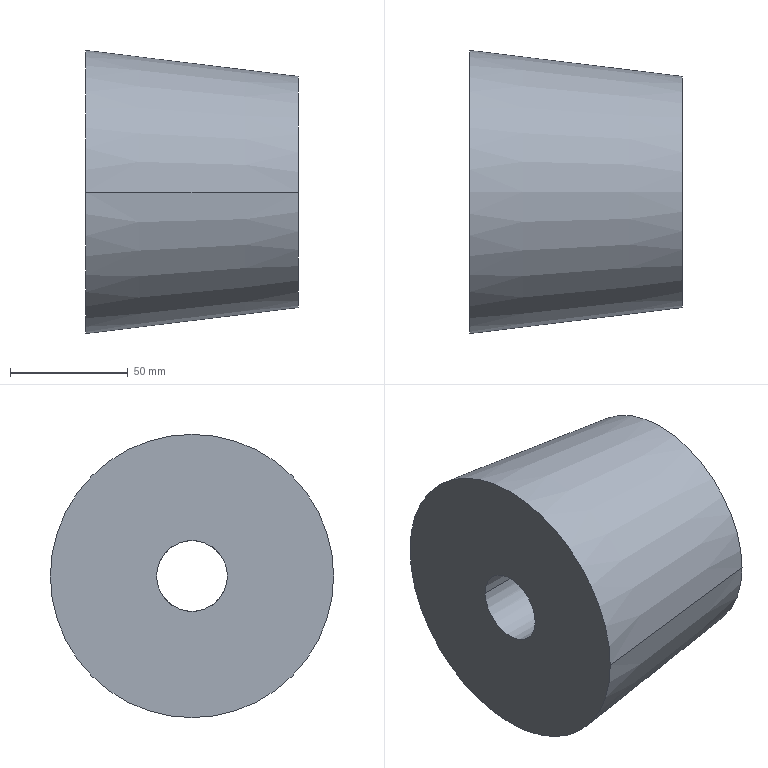Component | SolidWorks | SpacerBlock-1 | 1 solid | 8 faces | box 90 x 120 x 120 mm | volume 778299 mm3 | cylinder 4 | cone 2 | plane 2 | commonest cylinder face diameters 30 x4
build123d program:
from build123d import *

# Parameters (mm, degrees)
SKETCH1_R                    = 15
REPAIR_TIEBARPINHOLE30_DEPTH = 43.75
SKETCH2_R                    = 49.574
REPAIR_PADSEATTOHUB_DEPTH    = 5.084
REPAIR_PADSEATTOHUB_TAPER    = 7
SKETCH3_R                    = 15
REPAIR_PADSEATHOLE30_DEPTH   = 3.5


with BuildPart() as part:
    # Sketch1_2 → Revolve1 (revolve)
    with BuildSketch(Plane(origin=(0, 78.868, 0), x_dir=(1, 0, 0), z_dir=(0, 1, 0))):
        Polygon((-29.173, -0.08395), (-89.173, -0.08395), (-89.173, -85), (-39.6, -85), align=None)
    revolve(axis=Axis((-89.173, 78.868, 0.08395), (0, 0, 1)))

    # Sketch1 → Repair_TieBarPinHole30 (cut, symmetric)
    with BuildSketch(Plane.XY.offset(42.582)):
        with Locations((-89.173, 78.868)):
            Circle(SKETCH1_R)
    extrude(amount=REPAIR_TIEBARPINHOLE30_DEPTH, both=True, mode=Mode.SUBTRACT)

    # Sketch2 → Repair_PadSeatToHub (add)
    with BuildSketch(Plane.XY.offset(85)):
        with Locations((-89.173, 78.868)):
            Circle(SKETCH2_R)
    extrude(amount=REPAIR_PADSEATTOHUB_DEPTH, taper=REPAIR_PADSEATTOHUB_TAPER)

    # Sketch3 → Repair_PadSeatHole30 (cut, symmetric)
    with BuildSketch(Plane.XY.offset(87.416)):
        with Locations((-89.173, 78.868)):
            Circle(SKETCH3_R)
    extrude(amount=REPAIR_PADSEATHOLE30_DEPTH, both=True, mode=Mode.SUBTRACT)


solid = part.part

# Placed as in the assembly
solid = solid.moved(Location((-252.416, 1268.01, -86.763), (0, 90, 0)))
STEP:
#1=CARTESIAN_POINT('',(-6.591,52.436,0.09488));
#2=VERTEX_POINT('',#1);
#3=CARTESIAN_POINT('',(-6.591,53.617,0.09488));
#4=VERTEX_POINT('',#3);
#5=CARTESIAN_POINT('',(-6.591,52.436,0.09488));
#6=CARTESIAN_POINT('',(-6.591,52.436,0.01757));
#7=CARTESIAN_POINT('',(-6.591,52.452,-0.0597));
#8=CARTESIAN_POINT('',(-6.591,52.511,-0.2025));
#9=CARTESIAN_POINT('',(-6.591,52.554,-0.268));
#10=CARTESIAN_POINT('',(-6.591,52.664,-0.3774));
#11=CARTESIAN_POINT('',(-6.591,52.729,-0.4211));
#12=CARTESIAN_POINT('',(-6.591,52.872,-0.4803));
#13=CARTESIAN_POINT('',(-6.591,52.949,-0.4957));
#14=CARTESIAN_POINT('',(-6.591,53.104,-0.4957));
#15=CARTESIAN_POINT('',(-6.591,53.181,-0.4803));
#16=CARTESIAN_POINT('',(-6.591,53.324,-0.4211));
#17=CARTESIAN_POINT('',(-6.591,53.39,-0.3774));
#18=CARTESIAN_POINT('',(-6.591,53.499,-0.268));
#19=CARTESIAN_POINT('',(-6.591,53.543,-0.2025));
#20=CARTESIAN_POINT('',(-6.591,53.602,-0.0597));
#21=CARTESIAN_POINT('',(-6.591,53.617,0.01757));
#22=CARTESIAN_POINT('',(-6.591,53.617,0.09488));
#23=B_SPLINE_CURVE_WITH_KNOTS('',3,(#5,#6,#7,#8,#9,#10,#11,#12,#13,#14,#15,#16,#17,#18,#19,#20,#21,#22),.UNSPECIFIED.,.F.,.F.,(4,2,2,2,2,2,2,2,4),(0.5,0.5625,0.625,0.6875,0.75,0.8125,0.875,0.9375,1.),.UNSPECIFIED.);
#24=EDGE_CURVE('',#2,#4,#23,.T.);
#25=ORIENTED_EDGE('',*,*,#24,.F.);
#26=CARTESIAN_POINT('',(-6.391,52.436,0.09488));
#27=VERTEX_POINT('',#26);
#28=CARTESIAN_POINT('',(-6.634,52.436,0.09488));
#29=DIRECTION('',(1.,0.,0.));
#30=VECTOR('',#29,39.37);
#31=LINE('',#28,#30);
#32=EDGE_CURVE('',#2,#27,#31,.T.);
#33=ORIENTED_EDGE('',*,*,#32,.T.);
#34=CARTESIAN_POINT('',(-6.391,53.617,0.09488));
#35=VERTEX_POINT('',#34);
#36=CARTESIAN_POINT('',(-6.391,53.027,0.09488));
#37=DIRECTION('',(1.,0.,0.));
#38=DIRECTION('',(0.,1.,0.));
#39=AXIS2_PLACEMENT_3D('',#36,#37,#38);
#40=CIRCLE('',#39,0.5906);
#41=EDGE_CURVE('',#27,#35,#40,.T.);
#42=ORIENTED_EDGE('',*,*,#41,.T.);
#43=CARTESIAN_POINT('',(-6.634,53.617,0.09488));
#44=DIRECTION('',(1.,0.,0.));
#45=VECTOR('',#44,39.37);
#46=LINE('',#43,#45);
#47=EDGE_CURVE('',#4,#35,#46,.T.);
#48=ORIENTED_EDGE('',*,*,#47,.F.);
#49=EDGE_LOOP('',(#25,#33,#42,#48));
#50=FACE_OUTER_BOUND('',#49,.T.);
#51=CARTESIAN_POINT('',(-6.634,53.027,0.09488));
#52=DIRECTION('',(1.,0.,0.));
#53=DIRECTION('',(0.,1.,0.));
#54=AXIS2_PLACEMENT_3D('',#51,#52,#53);
#55=CYLINDRICAL_SURFACE('',#54,0.5906);
#56=ADVANCED_FACE('',(#50),#55,.F.);
#57=CARTESIAN_POINT('',(-9.934,53.617,0.09488));
#58=VERTEX_POINT('',#57);
#59=CARTESIAN_POINT('',(-9.934,52.436,0.09488));
#60=VERTEX_POINT('',#59);
#61=CARTESIAN_POINT('',(-9.934,53.027,0.09488));
#62=DIRECTION('',(-1.,0.,0.));
#63=DIRECTION('',(0.,-1.,0.));
#64=AXIS2_PLACEMENT_3D('',#61,#62,#63);
#65=CIRCLE('',#64,0.5906);
#66=EDGE_CURVE('',#58,#60,#65,.T.);
#67=ORIENTED_EDGE('',*,*,#66,.T.);
#68=CARTESIAN_POINT('',(-9.984,52.436,0.09488));
#69=DIRECTION('',(1.,0.,0.));
#70=VECTOR('',#69,39.37);
#71=LINE('',#68,#70);
#72=EDGE_CURVE('',#60,#2,#71,.T.);
#73=ORIENTED_EDGE('',*,*,#72,.T.);
#74=ORIENTED_EDGE('',*,*,#24,.T.);
#75=CARTESIAN_POINT('',(-9.984,53.617,0.09488));
#76=DIRECTION('',(1.,0.,0.));
#77=VECTOR('',#76,39.37);
#78=LINE('',#75,#77);
#79=EDGE_CURVE('',#58,#4,#78,.T.);
#80=ORIENTED_EDGE('',*,*,#79,.F.);
#81=EDGE_LOOP('',(#67,#73,#74,#80));
#82=FACE_OUTER_BOUND('',#81,.T.);
#83=CARTESIAN_POINT('',(-9.984,53.027,0.09488));
#84=DIRECTION('',(1.,0.,0.));
#85=DIRECTION('',(0.,1.,0.));
#86=AXIS2_PLACEMENT_3D('',#83,#84,#85);
#87=CYLINDRICAL_SURFACE('',#86,0.5906);
#88=ADVANCED_FACE('',(#82),#87,.F.);
#89=CARTESIAN_POINT('',(-6.391,54.954,0.09488));
#90=VERTEX_POINT('',#89);
#91=CARTESIAN_POINT('',(-6.391,51.1,0.09488));
#92=VERTEX_POINT('',#91);
#93=CARTESIAN_POINT('',(-6.391,53.027,0.09488));
#94=DIRECTION('',(1.,0.,0.));
#95=DIRECTION('',(0.,1.,0.));
#96=AXIS2_PLACEMENT_3D('',#93,#94,#95);
#97=CIRCLE('',#96,1.927);
#98=EDGE_CURVE('',#90,#92,#97,.T.);
#99=ORIENTED_EDGE('',*,*,#98,.F.);
#100=CARTESIAN_POINT('',(-9.934,55.389,0.09488));
#101=VERTEX_POINT('',#100);
#102=CARTESIAN_POINT('',(-6.591,54.978,0.09488));
#103=DIRECTION('',(-0.9925,0.1219,0.));
#104=VECTOR('',#103,39.37);
#105=LINE('',#102,#104);
#106=EDGE_CURVE('',#90,#101,#105,.T.);
#107=ORIENTED_EDGE('',*,*,#106,.T.);
#108=CARTESIAN_POINT('',(-9.934,50.664,0.09488));
#109=VERTEX_POINT('',#108);
#110=CARTESIAN_POINT('',(-9.934,53.027,0.09488));
#111=DIRECTION('',(1.,0.,0.));
#112=DIRECTION('',(0.,1.,0.));
#113=AXIS2_PLACEMENT_3D('',#110,#111,#112);
#114=CIRCLE('',#113,2.362);
#115=EDGE_CURVE('',#101,#109,#114,.T.);
#116=ORIENTED_EDGE('',*,*,#115,.T.);
#117=CARTESIAN_POINT('',(-6.591,51.075,0.09488));
#118=DIRECTION('',(-0.9925,-0.1219,0.));
#119=VECTOR('',#118,39.37);
#120=LINE('',#117,#119);
#121=EDGE_CURVE('',#92,#109,#120,.T.);
#122=ORIENTED_EDGE('',*,*,#121,.F.);
#123=EDGE_LOOP('',(#99,#107,#116,#122));
#124=FACE_OUTER_BOUND('',#123,.T.);
#125=CARTESIAN_POINT('',(-6.591,53.027,0.09488));
#126=DIRECTION('',(-1.,0.,0.));
#127=DIRECTION('',(0.,-1.,0.));
#128=AXIS2_PLACEMENT_3D('',#125,#126,#127);
#129=CONICAL_SURFACE('',#128,1.952,0.1222);
#130=ADVANCED_FACE('',(#124),#129,.T.);
#131=ORIENTED_EDGE('',*,*,#106,.F.);
#132=CARTESIAN_POINT('',(-6.391,53.027,0.09488));
#133=DIRECTION('',(1.,0.,0.));
#134=DIRECTION('',(0.,1.,0.));
#135=AXIS2_PLACEMENT_3D('',#132,#133,#134);
#136=CIRCLE('',#135,1.927);
#137=EDGE_CURVE('',#92,#90,#136,.T.);
#138=ORIENTED_EDGE('',*,*,#137,.F.);
#139=ORIENTED_EDGE('',*,*,#121,.T.);
#140=CARTESIAN_POINT('',(-9.934,53.027,0.09488));
#141=DIRECTION('',(1.,0.,0.));
#142=DIRECTION('',(0.,1.,0.));
#143=AXIS2_PLACEMENT_3D('',#140,#141,#142);
#144=CIRCLE('',#143,2.362);
#145=EDGE_CURVE('',#109,#101,#144,.T.);
#146=ORIENTED_EDGE('',*,*,#145,.T.);
#147=EDGE_LOOP('',(#131,#138,#139,#146));
#148=FACE_OUTER_BOUND('',#147,.T.);
#149=CARTESIAN_POINT('',(-6.591,53.027,0.09488));
#150=DIRECTION('',(-1.,0.,0.));
#151=DIRECTION('',(0.,-1.,0.));
#152=AXIS2_PLACEMENT_3D('',#149,#150,#151);
#153=CONICAL_SURFACE('',#152,1.952,0.1222);
#154=ADVANCED_FACE('',(#148),#153,.T.);
#155=ORIENTED_EDGE('',*,*,#66,.F.);
#156=CARTESIAN_POINT('',(-9.934,53.027,0.09488));
#157=DIRECTION('',(-1.,0.,0.));
#158=DIRECTION('',(0.,-1.,0.));
#159=AXIS2_PLACEMENT_3D('',#156,#157,#158);
#160=CIRCLE('',#159,0.5906);
#161=EDGE_CURVE('',#60,#58,#160,.T.);
#162=ORIENTED_EDGE('',*,*,#161,.F.);
#163=EDGE_LOOP('',(#155,#162));
#164=FACE_BOUND('',#163,.T.);
#165=ORIENTED_EDGE('',*,*,#145,.F.);
#166=ORIENTED_EDGE('',*,*,#115,.F.);
#167=EDGE_LOOP('',(#165,#166));
#168=FACE_OUTER_BOUND('',#167,.T.);
#169=CARTESIAN_POINT('',(-9.934,55.389,0.09488));
#170=DIRECTION('',(-1.,0.,0.));
#171=DIRECTION('',(0.,-1.,0.));
#172=AXIS2_PLACEMENT_3D('',#169,#170,#171);
#173=PLANE('',#172);
#174=ADVANCED_FACE('',(#164,#168),#173,.T.);
#175=ORIENTED_EDGE('',*,*,#72,.F.);
#176=ORIENTED_EDGE('',*,*,#161,.T.);
#177=ORIENTED_EDGE('',*,*,#79,.T.);
#178=CARTESIAN_POINT('',(-6.591,53.617,0.09488));
#179=CARTESIAN_POINT('',(-6.591,53.617,0.1722));
#180=CARTESIAN_POINT('',(-6.591,53.602,0.2495));
#181=CARTESIAN_POINT('',(-6.591,53.543,0.3923));
#182=CARTESIAN_POINT('',(-6.591,53.499,0.4578));
#183=CARTESIAN_POINT('',(-6.591,53.39,0.5671));
#184=CARTESIAN_POINT('',(-6.591,53.324,0.6109));
#185=CARTESIAN_POINT('',(-6.591,53.181,0.6701));
#186=CARTESIAN_POINT('',(-6.591,53.104,0.6854));
#187=CARTESIAN_POINT('',(-6.591,52.949,0.6854));
#188=CARTESIAN_POINT('',(-6.591,52.872,0.6701));
#189=CARTESIAN_POINT('',(-6.591,52.729,0.6109));
#190=CARTESIAN_POINT('',(-6.591,52.664,0.5671));
#191=CARTESIAN_POINT('',(-6.591,52.554,0.4578));
#192=CARTESIAN_POINT('',(-6.591,52.511,0.3923));
#193=CARTESIAN_POINT('',(-6.591,52.452,0.2495));
#194=CARTESIAN_POINT('',(-6.591,52.436,0.1722));
#195=CARTESIAN_POINT('',(-6.591,52.436,0.09488));
#196=B_SPLINE_CURVE_WITH_KNOTS('',3,(#178,#179,#180,#181,#182,#183,#184,#185,#186,#187,#188,#189,#190,#191,#192,#193,#194,#195),.UNSPECIFIED.,.F.,.F.,(4,2,2,2,2,2,2,2,4),(0.,0.0625,0.125,0.1875,0.25,0.3125,0.375,0.4375,0.5),.UNSPECIFIED.);
#197=EDGE_CURVE('',#4,#2,#196,.T.);
#198=ORIENTED_EDGE('',*,*,#197,.T.);
#199=EDGE_LOOP('',(#175,#176,#177,#198));
#200=FACE_OUTER_BOUND('',#199,.T.);
#201=CARTESIAN_POINT('',(-9.984,53.027,0.09488));
#202=DIRECTION('',(1.,0.,0.));
#203=DIRECTION('',(0.,1.,0.));
#204=AXIS2_PLACEMENT_3D('',#201,#202,#203);
#205=CYLINDRICAL_SURFACE('',#204,0.5906);
#206=ADVANCED_FACE('',(#200),#205,.F.);
#207=CARTESIAN_POINT('',(-6.391,53.027,0.09488));
#208=DIRECTION('',(1.,0.,0.));
#209=DIRECTION('',(0.,1.,0.));
#210=AXIS2_PLACEMENT_3D('',#207,#208,#209);
#211=CIRCLE('',#210,0.5906);
#212=EDGE_CURVE('',#35,#27,#211,.T.);
#213=ORIENTED_EDGE('',*,*,#212,.F.);
#214=ORIENTED_EDGE('',*,*,#41,.F.);
#215=EDGE_LOOP('',(#213,#214));
#216=FACE_BOUND('',#215,.T.);
#217=ORIENTED_EDGE('',*,*,#137,.T.);
#218=ORIENTED_EDGE('',*,*,#98,.T.);
#219=EDGE_LOOP('',(#217,#218));
#220=FACE_OUTER_BOUND('',#219,.T.);
#221=CARTESIAN_POINT('',(-6.391,53.027,0.09488));
#222=DIRECTION('',(1.,0.,0.));
#223=DIRECTION('',(0.,1.,0.));
#224=AXIS2_PLACEMENT_3D('',#221,#222,#223);
#225=PLANE('',#224);
#226=ADVANCED_FACE('',(#216,#220),#225,.T.);
#227=ORIENTED_EDGE('',*,*,#32,.F.);
#228=ORIENTED_EDGE('',*,*,#197,.F.);
#229=ORIENTED_EDGE('',*,*,#47,.T.);
#230=ORIENTED_EDGE('',*,*,#212,.T.);
#231=EDGE_LOOP('',(#227,#228,#229,#230));
#232=FACE_OUTER_BOUND('',#231,.T.);
#233=CARTESIAN_POINT('',(-6.634,53.027,0.09488));
#234=DIRECTION('',(1.,0.,0.));
#235=DIRECTION('',(0.,1.,0.));
#236=AXIS2_PLACEMENT_3D('',#233,#234,#235);
#237=CYLINDRICAL_SURFACE('',#236,0.5906);
#238=ADVANCED_FACE('',(#232),#237,.F.);
#239=CLOSED_SHELL('',(#56,#88,#130,#154,#174,#206,#226,#238));
#240=MANIFOLD_SOLID_BREP('',#239);
#241=CARTESIAN_POINT('',(0.,0.,0.));
#242=DIRECTION('',(0.,0.,1.));
#243=DIRECTION('',(1.,0.,0.));
#244=AXIS2_PLACEMENT_3D('',#241,#242,#243);
#245=(LENGTH_UNIT()NAMED_UNIT(*)SI_UNIT($,.METRE.));
#246=LENGTH_MEASURE_WITH_UNIT(LENGTH_MEASURE(0.0254),#245);
#247=DIMENSIONAL_EXPONENTS(1.,0.,0.,0.,0.,0.,0.);
#248=(CONVERSION_BASED_UNIT('',#246)LENGTH_UNIT()NAMED_UNIT(#247));
#249=UNCERTAINTY_MEASURE_WITH_UNIT(LENGTH_MEASURE(0.00001),#248,'','');
#250=(NAMED_UNIT(*)PLANE_ANGLE_UNIT()SI_UNIT($,.RADIAN.));
#251=(NAMED_UNIT(*)SI_UNIT($,.STERADIAN.)SOLID_ANGLE_UNIT());
#252=(GEOMETRIC_REPRESENTATION_CONTEXT(3)GLOBAL_UNCERTAINTY_ASSIGNED_CONTEXT((#249))GLOBAL_UNIT_ASSIGNED_CONTEXT((#248,#250,#251))REPRESENTATION_CONTEXT('',''));
#253=ADVANCED_BREP_SHAPE_REPRESENTATION('',(#240,#244),#252);
#254=COLOUR_RGB('',0.7922,0.8196,0.9333);
#255=FILL_AREA_STYLE_COLOUR('',#254);
#256=FILL_AREA_STYLE('',(#255));
#257=SURFACE_STYLE_FILL_AREA(#256);
#258=SURFACE_SIDE_STYLE('',(#257));
#259=SURFACE_STYLE_USAGE(.BOTH.,#258);
#260=PRESENTATION_STYLE_ASSIGNMENT((#259));
#261=STYLED_ITEM('',(#260),#240);
#262=(LENGTH_UNIT()NAMED_UNIT(*)SI_UNIT($,.METRE.));
#263=LENGTH_MEASURE_WITH_UNIT(LENGTH_MEASURE(0.0254),#262);
#264=DIMENSIONAL_EXPONENTS(1.,0.,0.,0.,0.,0.,0.);
#265=(CONVERSION_BASED_UNIT('',#263)LENGTH_UNIT()NAMED_UNIT(#264));
#266=UNCERTAINTY_MEASURE_WITH_UNIT(LENGTH_MEASURE(0.00001),#265,'','');
#267=(NAMED_UNIT(*)PLANE_ANGLE_UNIT()SI_UNIT($,.RADIAN.));
#268=(NAMED_UNIT(*)SI_UNIT($,.STERADIAN.)SOLID_ANGLE_UNIT());
#269=(GEOMETRIC_REPRESENTATION_CONTEXT(3)GLOBAL_UNCERTAINTY_ASSIGNED_CONTEXT((#266))GLOBAL_UNIT_ASSIGNED_CONTEXT((#265,#267,#268))REPRESENTATION_CONTEXT('',''));
#270=MECHANICAL_DESIGN_GEOMETRIC_PRESENTATION_REPRESENTATION('',(#261),#269);
#271=PRESENTATION_LAYER_ASSIGNMENT('','',(#261));